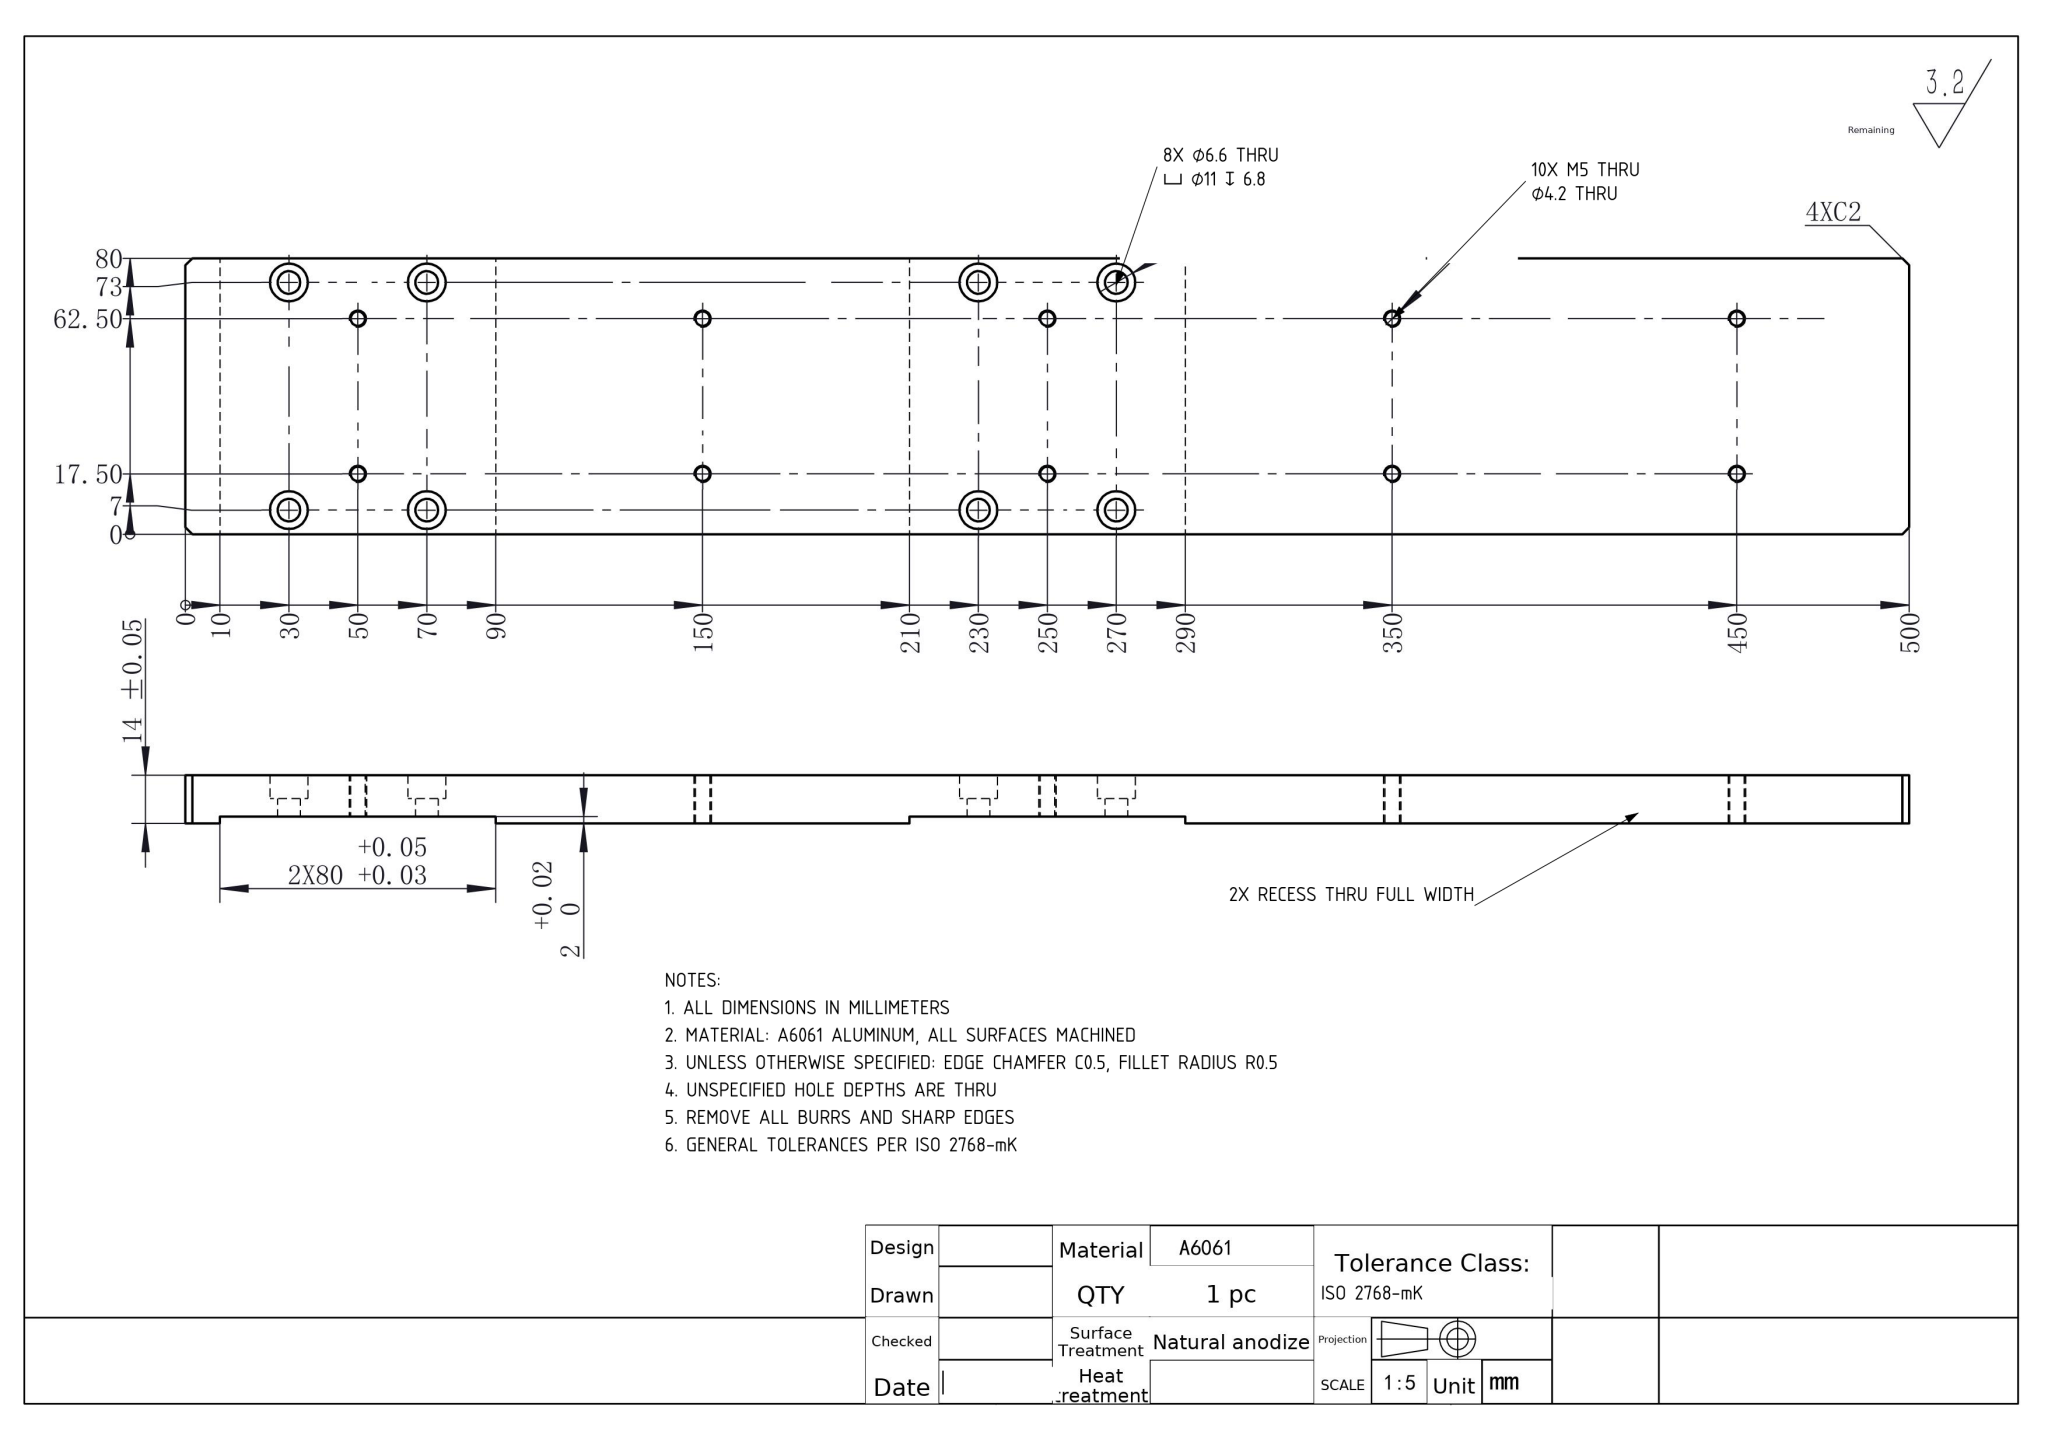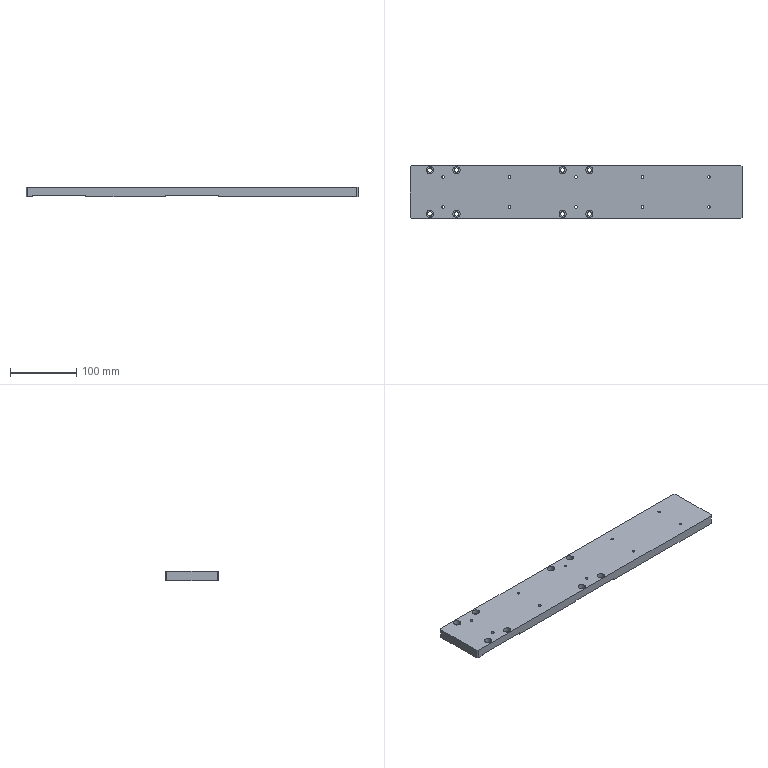Part | NX | mm | 1 solid | 78 faces | box 500 x 80 x 14 mm | volume 525866 mm3 | cylinder 52 | plane 26 | commonest cylinder face diameters 4.2 x20 11 x16 6.6 x16